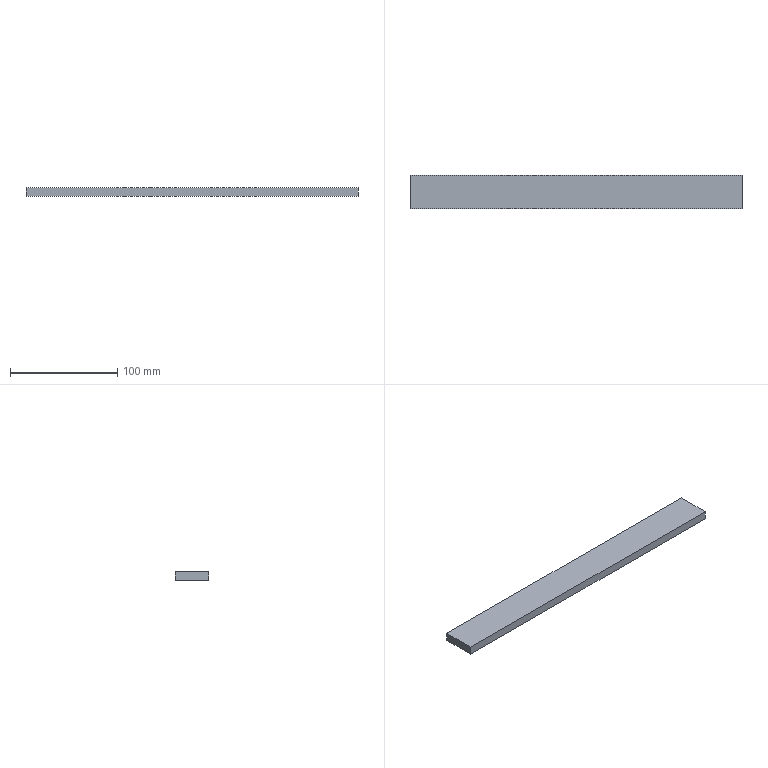CAM job | Mastercam | mm | 2 operations | part box 310 x 48.92 x 8
1. Drill/Counterbore | 12 - 12 定位钻
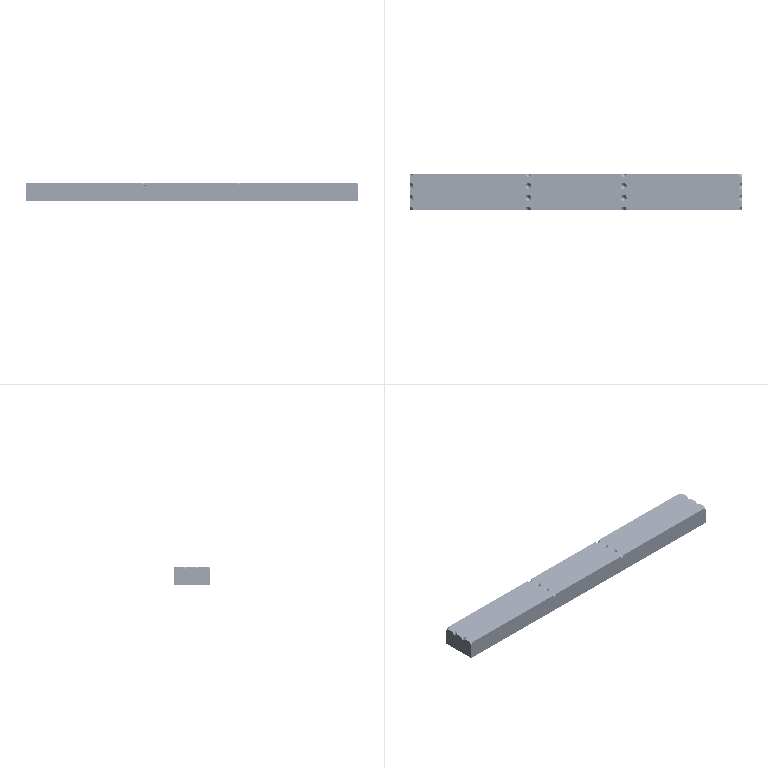2. Peck Drill | 20 - 3.5 钻头